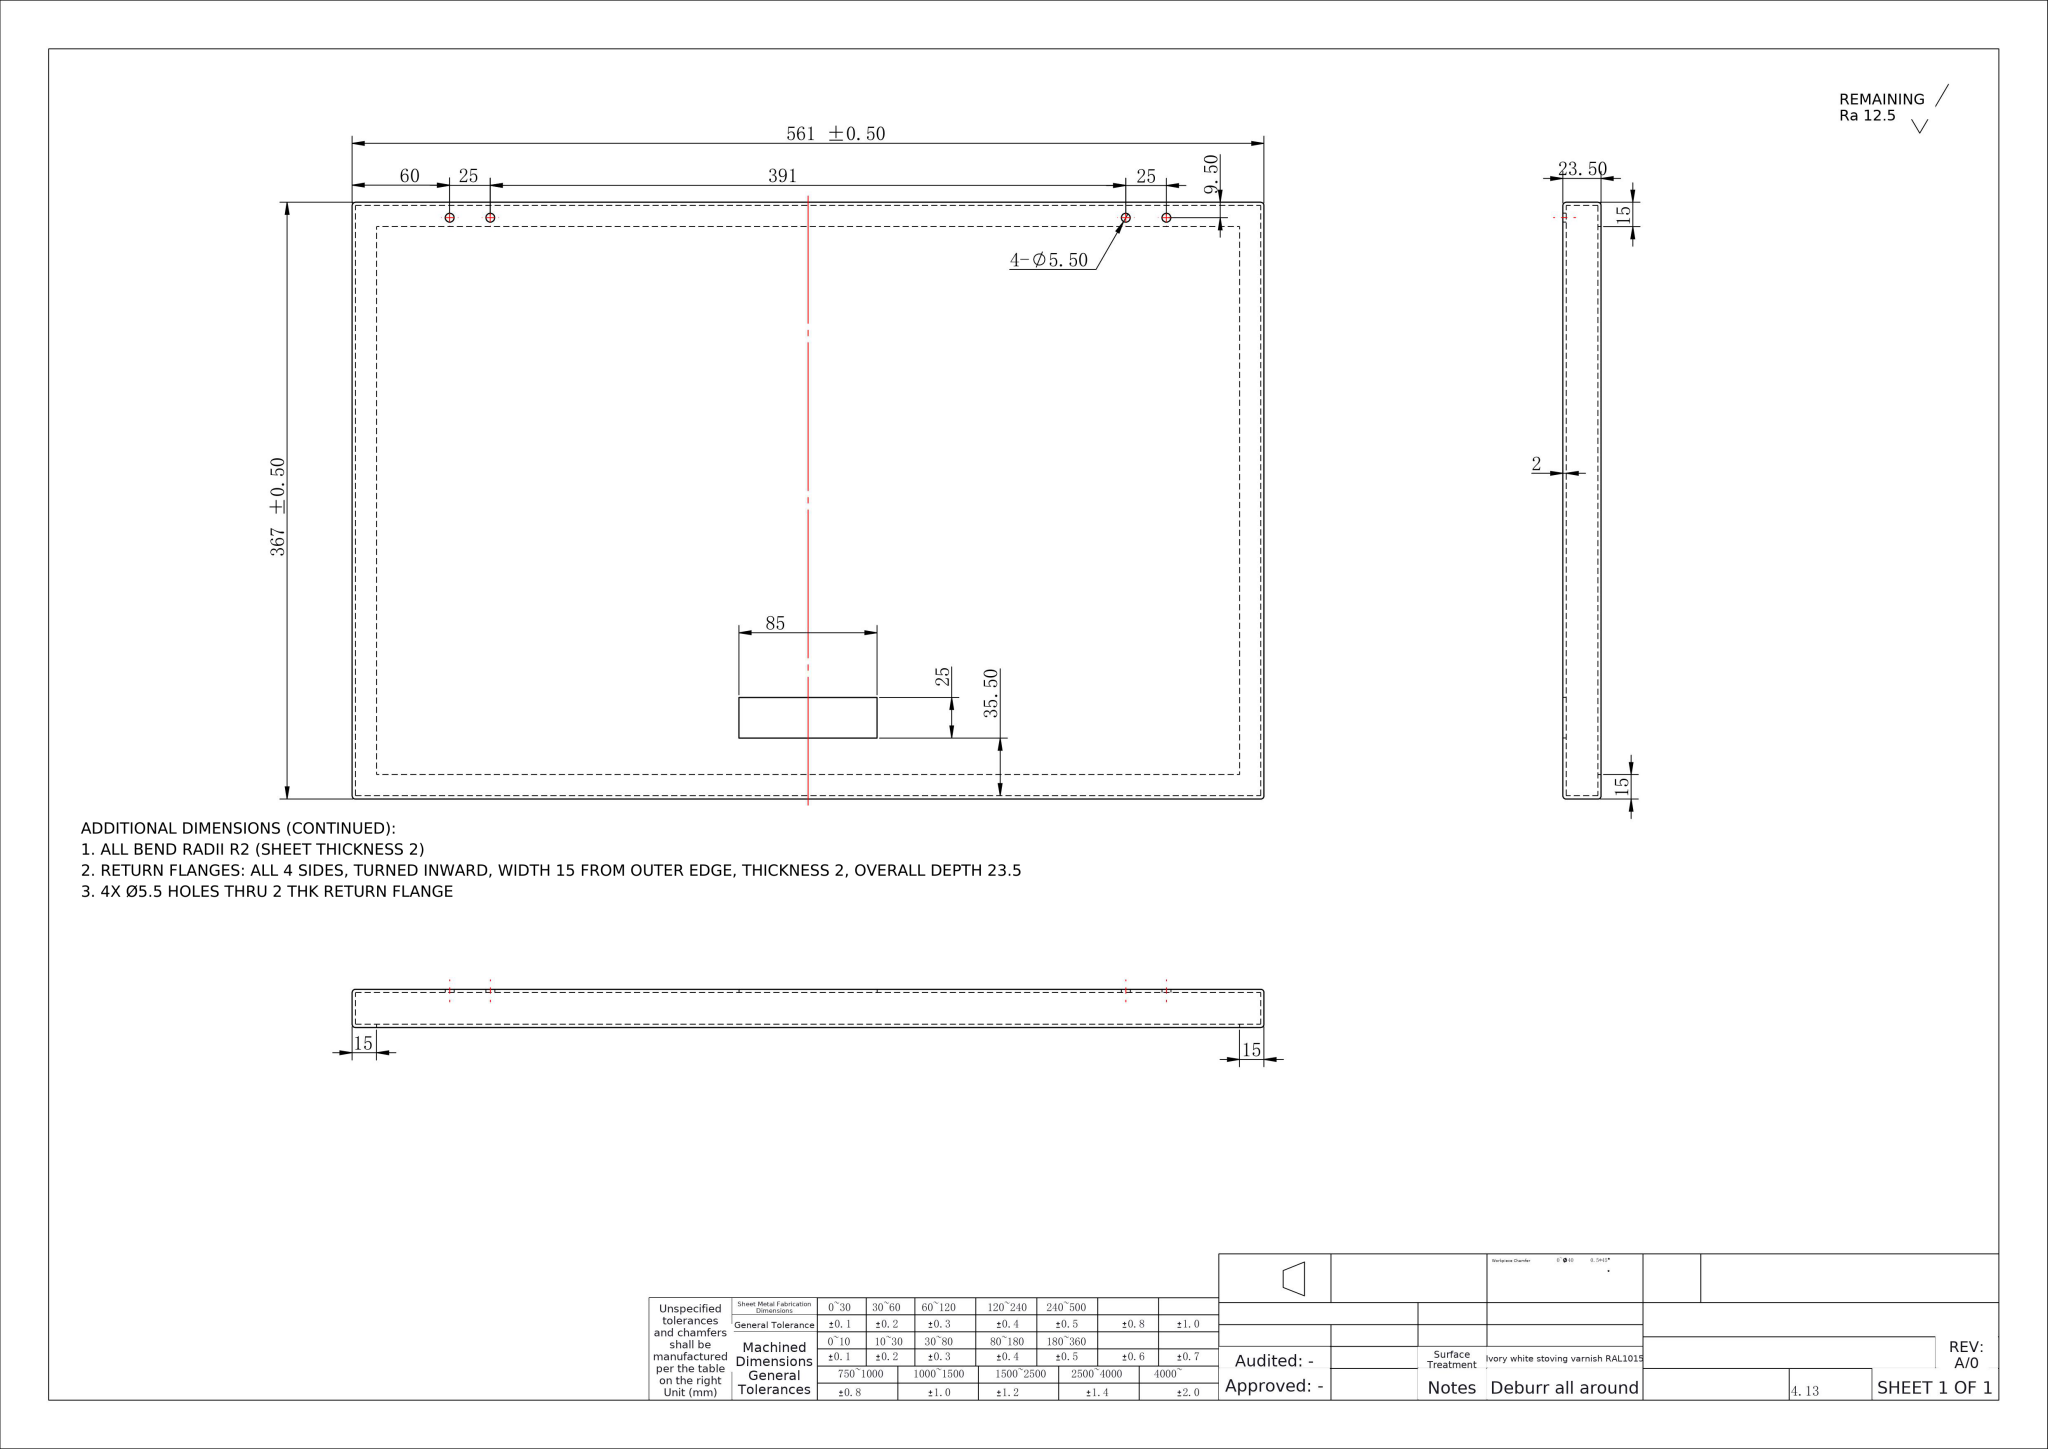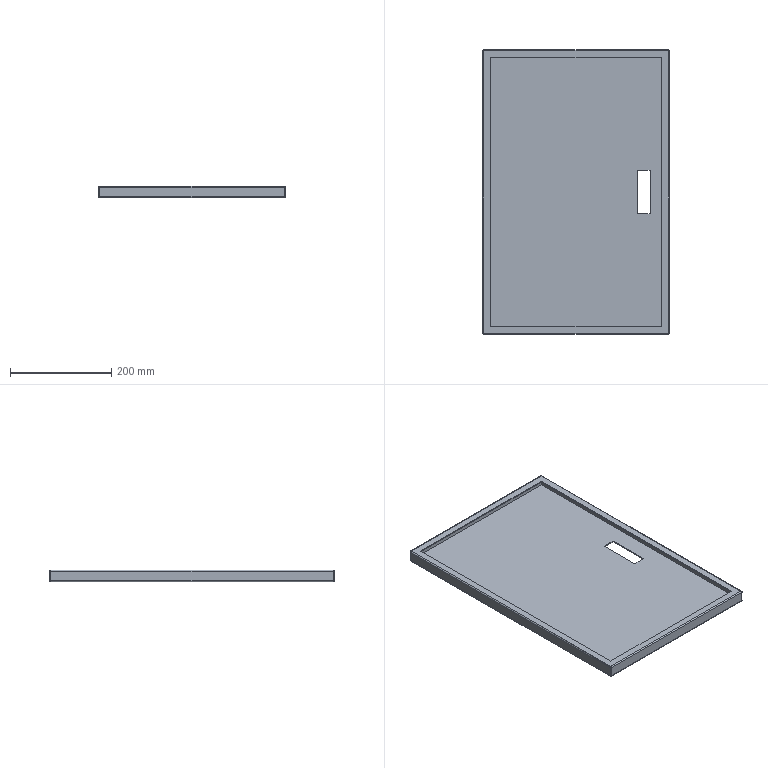Part | NX | mm | 1 solid | 48 faces | box 367 x 561 x 23.5 mm | volume 530030 mm3 | cylinder 20 | plane 20 | sphere 8 | commonest cylinder face diameters 4 x12 5.5 x8